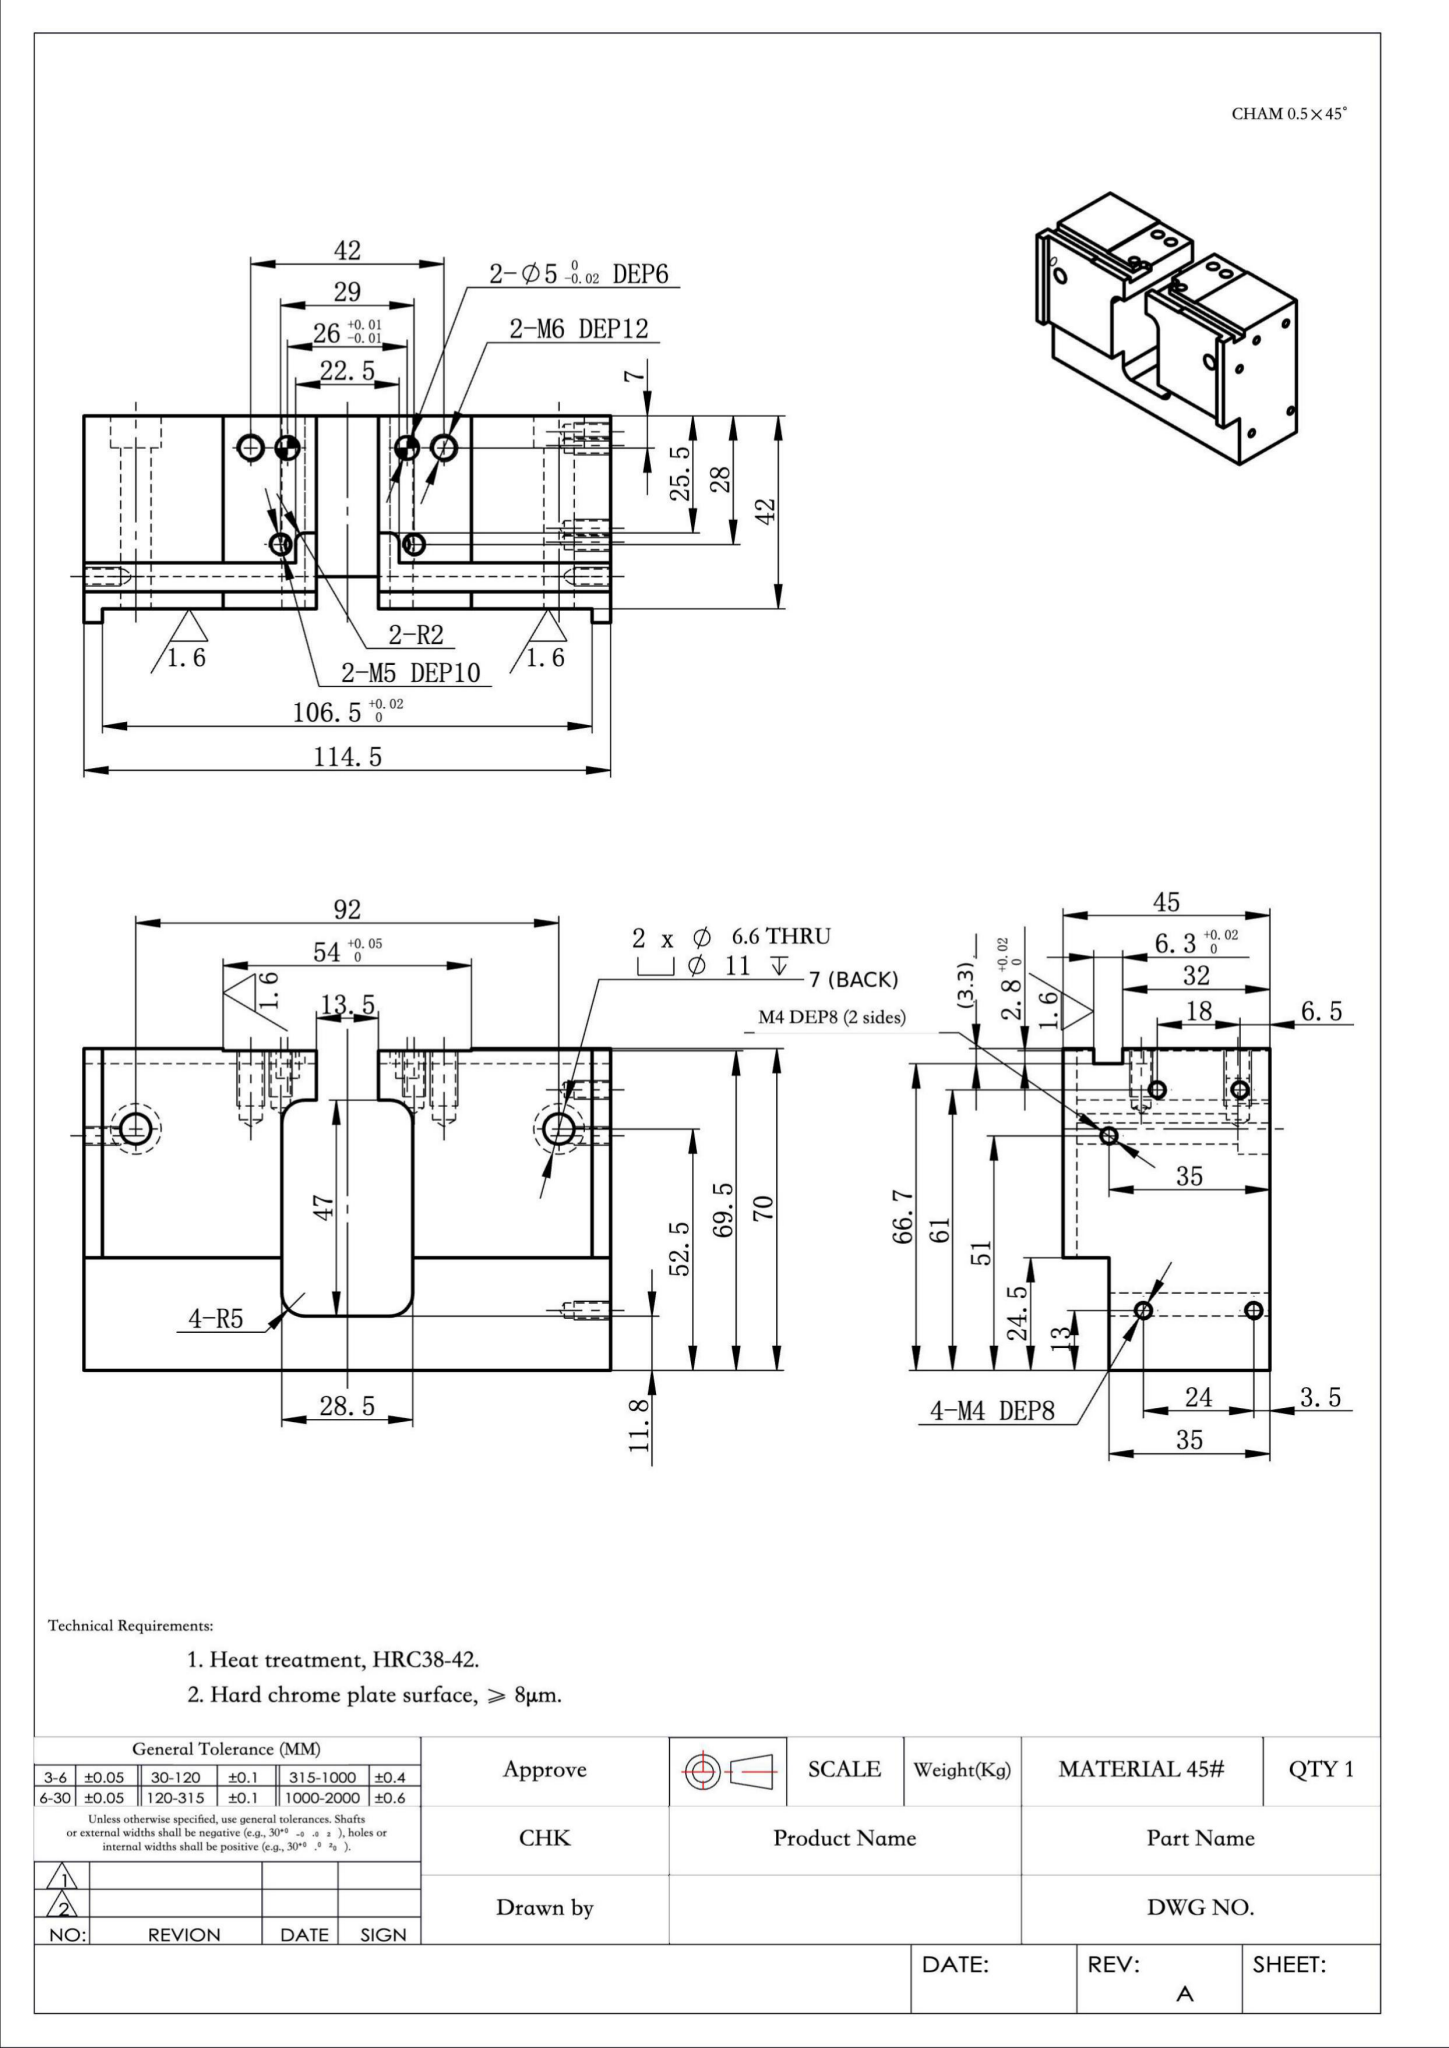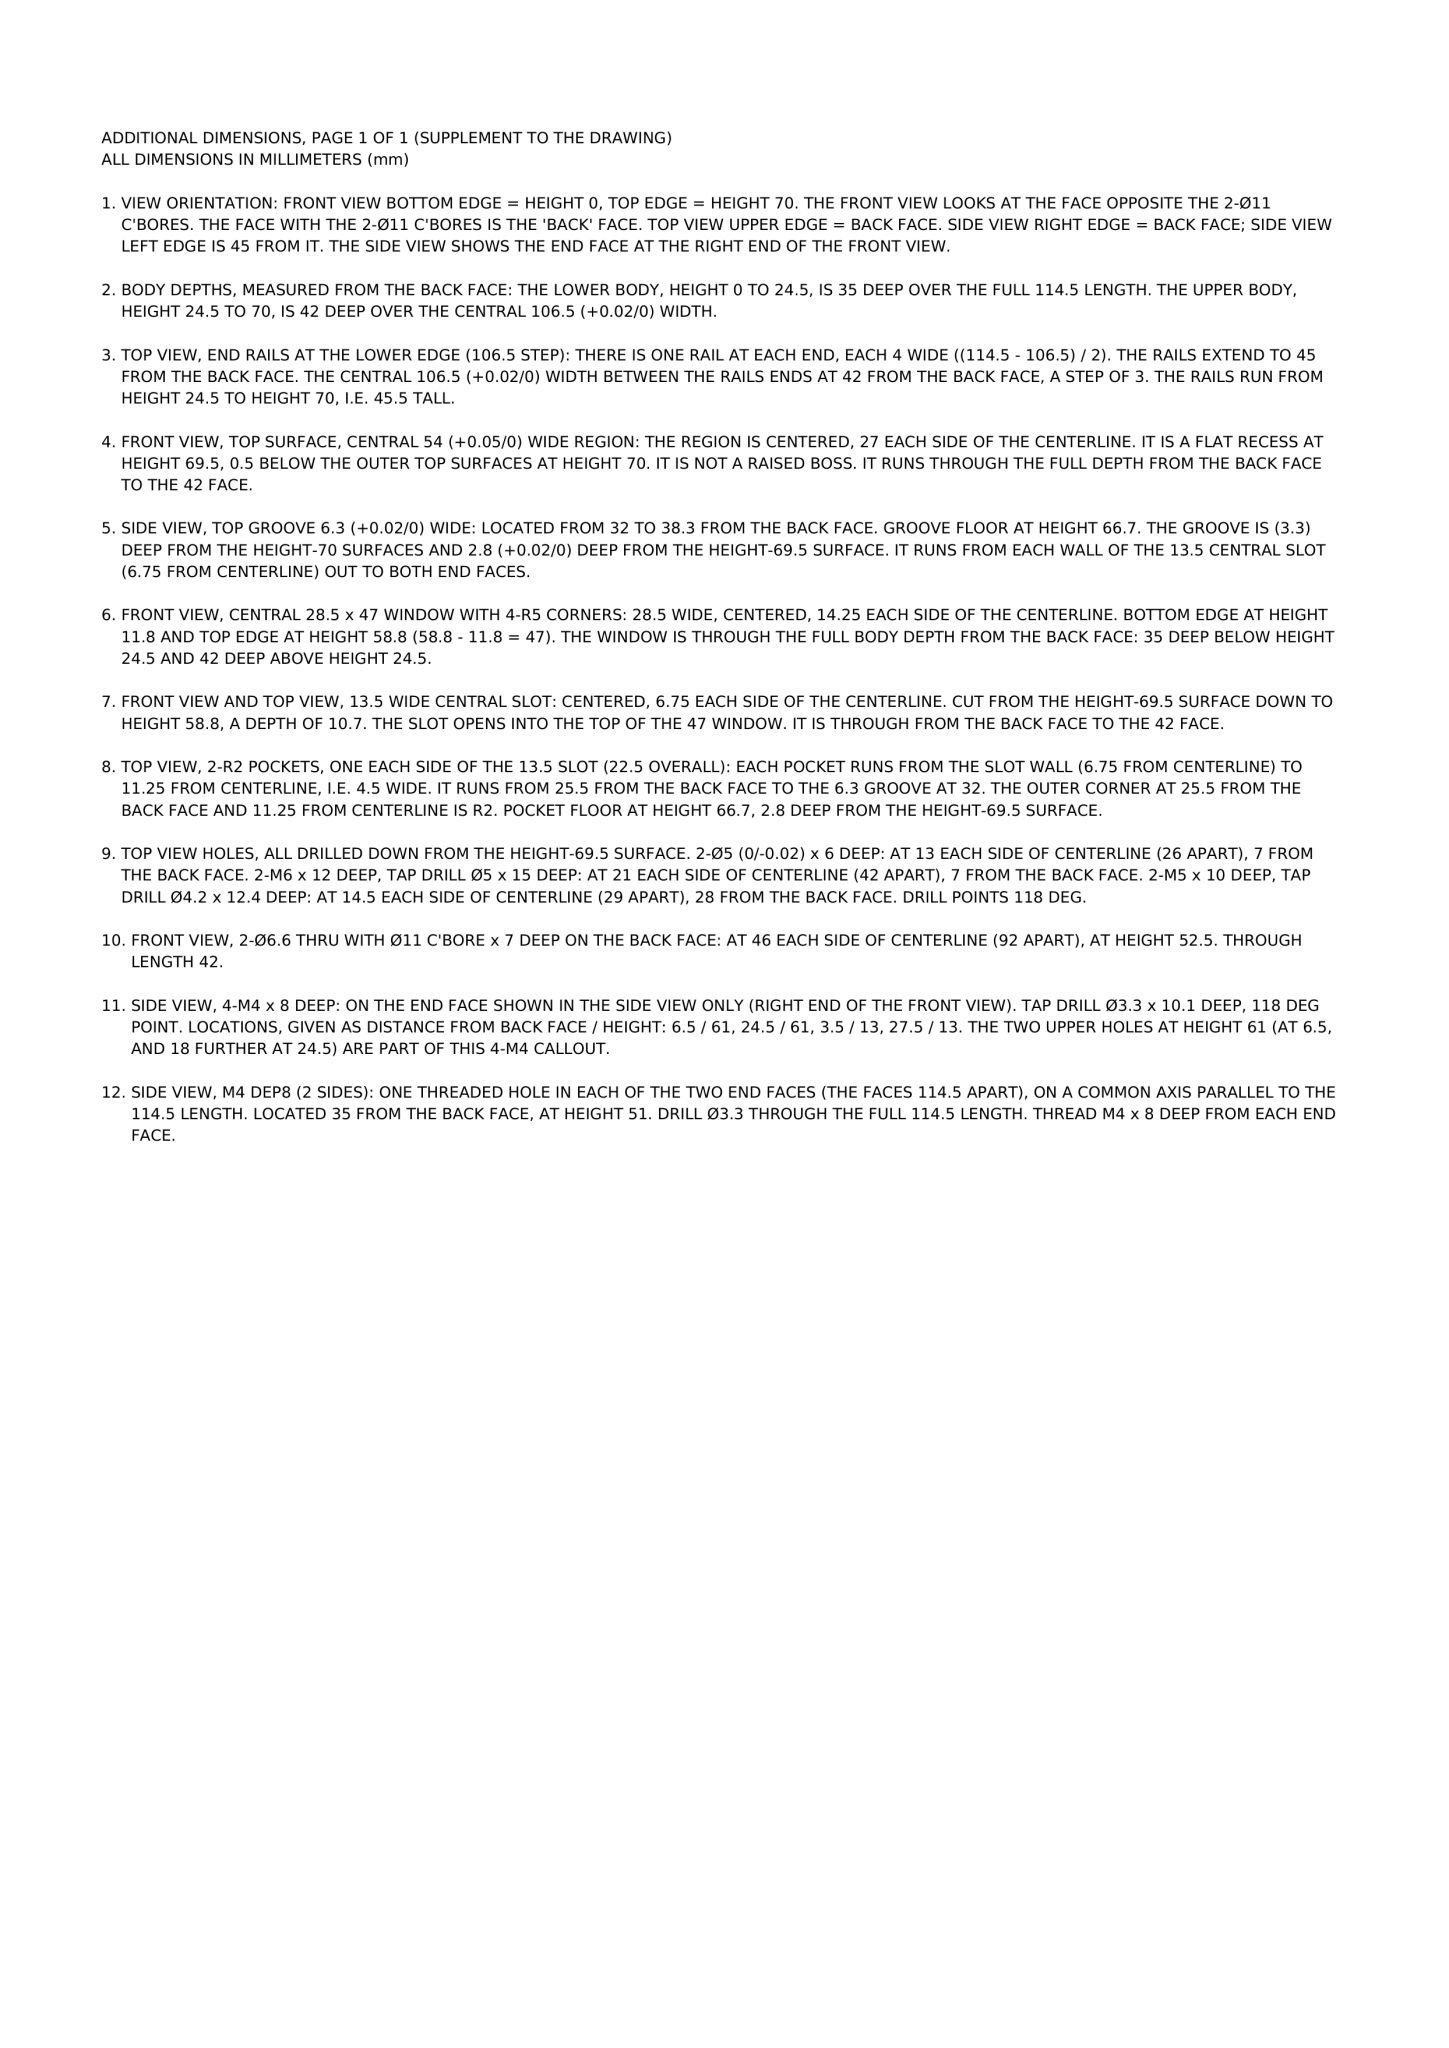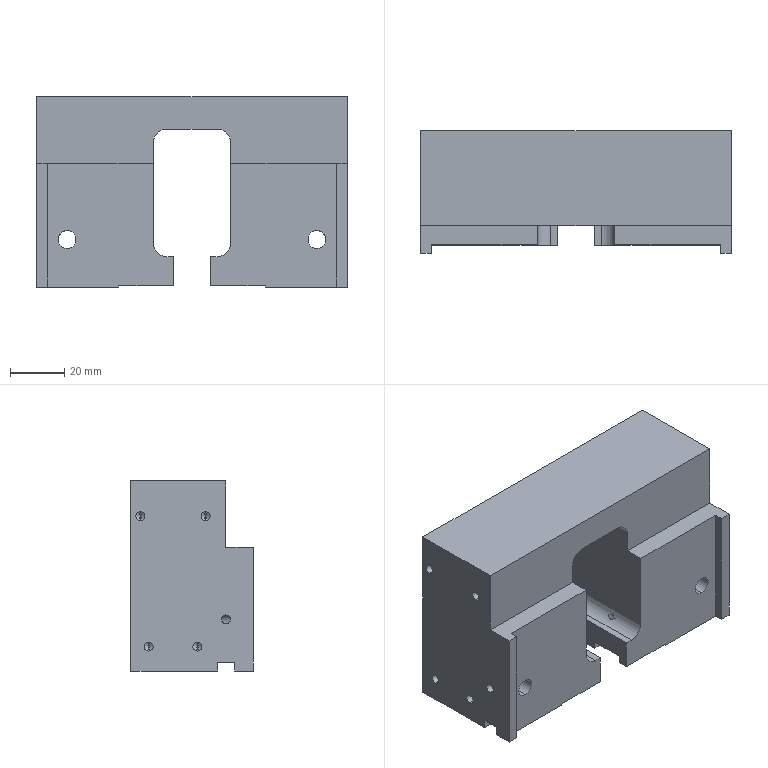Part | NX | mm | 1 solid | 103 faces | box 114.5 x 45 x 70 mm | volume 250429 mm3 | plane 46 | cylinder 38 | cone 19 | commonest cylinder face diameters 3.3 x12 5 x8 4.2 x4 11 x4 6.6 x4 10 x4 4 x2